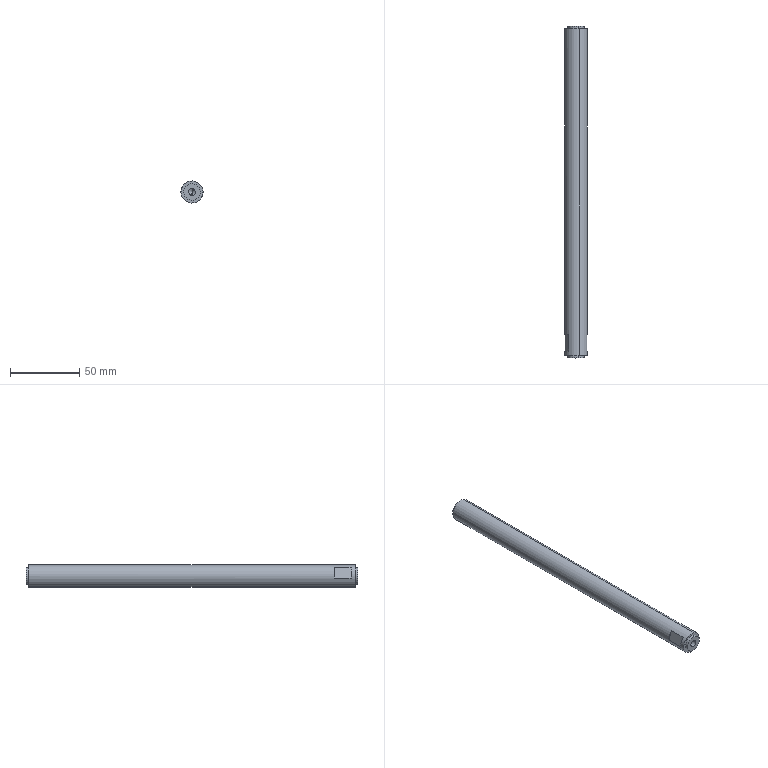Component | SolidWorks | F01AE00111-A2014-1 | 1 solid | 24 faces | box 16 x 240 x 16 mm | volume 47169 mm3 | cylinder 10 | plane 10 | cone 4 | commonest cylinder face diameters 5 x4 12 x4 16 x2 | material Hard Chrome Plated Rod
build123d program:
from build123d import *

# Parameters (mm, degrees)
SKETCH1_R             = 8
BOSS_EXTRUDE1_DEPTH   = 240
CHAMFER1_SIZE         = 1
M6_TAPPED_HOLE1_D     = 5
M6_TAPPED_HOLE1_DEPTH = 15
M6_TAPPED_HOLE1_TIP   = 1.502
SKETCH4_R             = 10.068
SKETCH4_R_2           = 6
CUT_EXTRUDE1_DEPTH    = 2
M6_TAPPED_HOLE2_D     = 5
M6_TAPPED_HOLE2_DEPTH = 15
M6_TAPPED_HOLE2_TIP   = 1.502
SKETCH7_W             = 3.867
SKETCH7_H             = 17.751
SKETCH7_W_2           = 7.143
SKETCH7_H_2           = 17.096
CUT_EXTRUDE2_DEPTH    = 12
SKETCH8_OUTSIDE_W     = 66.212
SKETCH8_OUTSIDE_H     = 66.212
SKETCH8_OUTSIDE_R     = 6
CUT_EXTRUDE3_DEPTH    = 2


with BuildPart() as part:
    # Sketch1 → Boss-Extrude1 (new body)
    with BuildSketch(Plane(origin=(0, 0, 0), x_dir=(1, 0, 0), z_dir=(0, 1, 0))):
        with Locations(Location((0, 0, 0), (0, 0, 270))):
            Circle(SKETCH1_R)
    extrude(amount=BOSS_EXTRUDE1_DEPTH)

    # Chamfer1
    chamfer1_edges = [part.edges().sort_by_distance(p)[0] for p in [
        (0, 0, -8),
        (0, 240, -8),
    ]]
    chamfer(chamfer1_edges, length=CHAMFER1_SIZE)

    # M6 Tapped Hole1
    with Locations(Plane(origin=(0, 240, 0), x_dir=(1, 0, 0), z_dir=(0, 1, 0))):
        with Locations((0, 0)):
            Hole(M6_TAPPED_HOLE1_D / 2, depth=M6_TAPPED_HOLE1_DEPTH)
            with Locations((0, 0, -(M6_TAPPED_HOLE1_DEPTH + M6_TAPPED_HOLE1_TIP / 2))):  # 118° drill point
                Cone(0, M6_TAPPED_HOLE1_D / 2, M6_TAPPED_HOLE1_TIP, mode=Mode.SUBTRACT)

    # Sketch4 → Cut-Extrude1 (cut)
    with BuildSketch(Plane(origin=(0, 240, 0), x_dir=(1, 0, 0), z_dir=(0, 1, 0))):
        Circle(SKETCH4_R)
        with Locations(Location((0, 0, 0), (0, 0, 270))):
            Circle(SKETCH4_R_2, mode=Mode.SUBTRACT)
    extrude(amount=-CUT_EXTRUDE1_DEPTH, mode=Mode.SUBTRACT)

    # M6 Tapped Hole2
    with Locations(Plane(origin=(0, 0, 0), x_dir=(-1, 0, 0), z_dir=(0, -1, 0))):
        with Locations((0, 0)):
            Hole(M6_TAPPED_HOLE2_D / 2, depth=M6_TAPPED_HOLE2_DEPTH)
            with Locations((0, 0, -(M6_TAPPED_HOLE2_DEPTH + M6_TAPPED_HOLE2_TIP / 2))):  # 118° drill point
                Cone(0, M6_TAPPED_HOLE2_D / 2, M6_TAPPED_HOLE2_TIP, mode=Mode.SUBTRACT)

    # Sketch7 → Cut-Extrude2 (cut)
    with BuildSketch(Plane(origin=(0, 5, 0), x_dir=(-1, 0, 0), z_dir=(0, -1, 0))):
        with Locations((-8.934, -0.05283)):
            Rectangle(SKETCH7_W, SKETCH7_H)
        with Locations((10.571, -0.2958)):
            Rectangle(SKETCH7_W_2, SKETCH7_H_2)
    extrude(amount=-CUT_EXTRUDE2_DEPTH, mode=Mode.SUBTRACT)

    # Sketch8 outside → Cut-Extrude3 (cut)
    with BuildSketch(Plane.XZ):
        Rectangle(SKETCH8_OUTSIDE_W, SKETCH8_OUTSIDE_H)
        with Locations(Location((0, 0, 0), (0, 0, 90))):
            Circle(SKETCH8_OUTSIDE_R, mode=Mode.SUBTRACT)
    extrude(amount=-CUT_EXTRUDE3_DEPTH, mode=Mode.SUBTRACT)


solid = part.part

# Placed as in the assembly
solid = solid.moved(Location((-84.852, -192.452, -211.475), (0, 18.481, 0)))
STEP:
#1=CARTESIAN_POINT('',(-3.309,-6.986,-8.232));
#2=VERTEX_POINT('',#1);
#3=CARTESIAN_POINT('',(-3.372,-6.986,-8.419));
#4=VERTEX_POINT('',#3);
#5=CARTESIAN_POINT('',(-3.341,-6.986,-8.326));
#6=DIRECTION('',(0.,-1.,0.));
#7=DIRECTION('',(-0.317,0.,-0.9484));
#8=AXIS2_PLACEMENT_3D('',#5,#6,#7);
#9=CIRCLE('',#8,0.09843);
#10=EDGE_CURVE('',#2,#4,#9,.T.);
#11=ORIENTED_EDGE('',*,*,#10,.F.);
#12=CARTESIAN_POINT('',(-3.309,-7.577,-8.232));
#13=VERTEX_POINT('',#12);
#14=CARTESIAN_POINT('',(-3.309,-7.577,-8.232));
#15=DIRECTION('',(0.,-1.,0.));
#16=VECTOR('',#15,39.37);
#17=LINE('',#14,#16);
#18=EDGE_CURVE('',#2,#13,#17,.T.);
#19=ORIENTED_EDGE('',*,*,#18,.T.);
#20=CARTESIAN_POINT('',(-3.372,-7.577,-8.419));
#21=VERTEX_POINT('',#20);
#22=CARTESIAN_POINT('',(-3.341,-7.577,-8.326));
#23=DIRECTION('',(0.,-1.,0.));
#24=DIRECTION('',(-0.317,0.,-0.9484));
#25=AXIS2_PLACEMENT_3D('',#22,#23,#24);
#26=CIRCLE('',#25,0.09843);
#27=EDGE_CURVE('',#13,#21,#26,.T.);
#28=ORIENTED_EDGE('',*,*,#27,.T.);
#29=CARTESIAN_POINT('',(-3.372,-7.577,-8.419));
#30=DIRECTION('',(0.,-1.,0.));
#31=VECTOR('',#30,39.37);
#32=LINE('',#29,#31);
#33=EDGE_CURVE('',#4,#21,#32,.T.);
#34=ORIENTED_EDGE('',*,*,#33,.F.);
#35=EDGE_LOOP('',(#11,#19,#28,#34));
#36=FACE_OUTER_BOUND('',#35,.T.);
#37=CARTESIAN_POINT('',(-3.341,-7.577,-8.326));
#38=DIRECTION('',(0.,-1.,0.));
#39=DIRECTION('',(-0.317,0.,-0.9484));
#40=AXIS2_PLACEMENT_3D('',#37,#38,#39);
#41=CYLINDRICAL_SURFACE('',#40,0.09843);
#42=ADVANCED_FACE('',(#36),#41,.F.);
#43=CARTESIAN_POINT('',(-3.341,-6.927,-8.326));
#44=VERTEX_POINT('',#43);
#45=CARTESIAN_POINT('',(-3.372,-6.986,-8.419));
#46=DIRECTION('',(-0.2717,-0.515,-0.813));
#47=VECTOR('',#46,39.37);
#48=LINE('',#45,#47);
#49=EDGE_CURVE('',#44,#4,#48,.T.);
#50=ORIENTED_EDGE('',*,*,#49,.F.);
#51=CARTESIAN_POINT('',(-3.309,-6.986,-8.232));
#52=DIRECTION('',(0.2717,-0.515,0.813));
#53=VECTOR('',#52,39.37);
#54=LINE('',#51,#53);
#55=EDGE_CURVE('',#44,#2,#54,.T.);
#56=ORIENTED_EDGE('',*,*,#55,.T.);
#57=ORIENTED_EDGE('',*,*,#10,.T.);
#58=EDGE_LOOP('',(#50,#56,#57));
#59=FACE_OUTER_BOUND('',#58,.T.);
#60=CARTESIAN_POINT('',(-3.341,-6.986,-8.326));
#61=DIRECTION('',(0.,-1.,0.));
#62=DIRECTION('',(-0.317,0.,-0.9484));
#63=AXIS2_PLACEMENT_3D('',#60,#61,#62);
#64=CONICAL_SURFACE('',#63,0.09843,1.03);
#65=ADVANCED_FACE('',(#59),#64,.F.);
#66=CARTESIAN_POINT('',(-3.416,-7.498,-8.55));
#67=VERTEX_POINT('',#66);
#68=CARTESIAN_POINT('',(-3.266,-7.498,-8.102));
#69=VERTEX_POINT('',#68);
#70=CARTESIAN_POINT('',(-3.341,-7.498,-8.326));
#71=DIRECTION('',(0.,-1.,0.));
#72=DIRECTION('',(-0.317,0.,-0.9484));
#73=AXIS2_PLACEMENT_3D('',#70,#71,#72);
#74=CIRCLE('',#73,0.2362);
#75=EDGE_CURVE('',#67,#69,#74,.T.);
#76=ORIENTED_EDGE('',*,*,#75,.T.);
#77=CARTESIAN_POINT('',(-3.266,-7.577,-8.102));
#78=VERTEX_POINT('',#77);
#79=CARTESIAN_POINT('',(-3.266,-7.498,-8.102));
#80=DIRECTION('',(0.,-1.,0.));
#81=VECTOR('',#80,39.37);
#82=LINE('',#79,#81);
#83=EDGE_CURVE('',#69,#78,#82,.T.);
#84=ORIENTED_EDGE('',*,*,#83,.T.);
#85=CARTESIAN_POINT('',(-3.416,-7.577,-8.55));
#86=VERTEX_POINT('',#85);
#87=CARTESIAN_POINT('',(-3.341,-7.577,-8.326));
#88=DIRECTION('',(0.,-1.,0.));
#89=DIRECTION('',(-0.317,0.,-0.9484));
#90=AXIS2_PLACEMENT_3D('',#87,#88,#89);
#91=CIRCLE('',#90,0.2362);
#92=EDGE_CURVE('',#86,#78,#91,.T.);
#93=ORIENTED_EDGE('',*,*,#92,.F.);
#94=CARTESIAN_POINT('',(-3.416,-7.498,-8.55));
#95=DIRECTION('',(0.,-1.,0.));
#96=VECTOR('',#95,39.37);
#97=LINE('',#94,#96);
#98=EDGE_CURVE('',#67,#86,#97,.T.);
#99=ORIENTED_EDGE('',*,*,#98,.F.);
#100=EDGE_LOOP('',(#76,#84,#93,#99));
#101=FACE_OUTER_BOUND('',#100,.T.);
#102=CARTESIAN_POINT('',(-3.341,-7.498,-8.326));
#103=DIRECTION('',(0.,-1.,0.));
#104=DIRECTION('',(-0.317,0.,-0.9484));
#105=AXIS2_PLACEMENT_3D('',#102,#103,#104);
#106=CYLINDRICAL_SURFACE('',#105,0.2362);
#107=ADVANCED_FACE('',(#101),#106,.T.);
#108=CARTESIAN_POINT('',(-3.372,1.281,-8.419));
#109=VERTEX_POINT('',#108);
#110=CARTESIAN_POINT('',(-3.309,1.281,-8.232));
#111=VERTEX_POINT('',#110);
#112=CARTESIAN_POINT('',(-3.341,1.281,-8.326));
#113=DIRECTION('',(0.,1.,0.));
#114=DIRECTION('',(0.317,0.,0.9484));
#115=AXIS2_PLACEMENT_3D('',#112,#113,#114);
#116=CIRCLE('',#115,0.09843);
#117=EDGE_CURVE('',#109,#111,#116,.T.);
#118=ORIENTED_EDGE('',*,*,#117,.F.);
#119=CARTESIAN_POINT('',(-3.372,1.872,-8.419));
#120=VERTEX_POINT('',#119);
#121=CARTESIAN_POINT('',(-3.372,1.872,-8.419));
#122=DIRECTION('',(0.,1.,0.));
#123=VECTOR('',#122,39.37);
#124=LINE('',#121,#123);
#125=EDGE_CURVE('',#109,#120,#124,.T.);
#126=ORIENTED_EDGE('',*,*,#125,.T.);
#127=CARTESIAN_POINT('',(-3.309,1.872,-8.232));
#128=VERTEX_POINT('',#127);
#129=CARTESIAN_POINT('',(-3.341,1.872,-8.326));
#130=DIRECTION('',(0.,1.,0.));
#131=DIRECTION('',(0.317,0.,0.9484));
#132=AXIS2_PLACEMENT_3D('',#129,#130,#131);
#133=CIRCLE('',#132,0.09843);
#134=EDGE_CURVE('',#120,#128,#133,.T.);
#135=ORIENTED_EDGE('',*,*,#134,.T.);
#136=CARTESIAN_POINT('',(-3.309,1.872,-8.232));
#137=DIRECTION('',(0.,1.,0.));
#138=VECTOR('',#137,39.37);
#139=LINE('',#136,#138);
#140=EDGE_CURVE('',#111,#128,#139,.T.);
#141=ORIENTED_EDGE('',*,*,#140,.F.);
#142=EDGE_LOOP('',(#118,#126,#135,#141));
#143=FACE_OUTER_BOUND('',#142,.T.);
#144=CARTESIAN_POINT('',(-3.341,1.872,-8.326));
#145=DIRECTION('',(0.,1.,0.));
#146=DIRECTION('',(0.317,0.,0.9484));
#147=AXIS2_PLACEMENT_3D('',#144,#145,#146);
#148=CYLINDRICAL_SURFACE('',#147,0.09843);
#149=ADVANCED_FACE('',(#143),#148,.F.);
#150=CARTESIAN_POINT('',(-3.341,1.222,-8.326));
#151=VERTEX_POINT('',#150);
#152=CARTESIAN_POINT('',(-3.309,1.281,-8.232));
#153=DIRECTION('',(0.2717,0.515,0.813));
#154=VECTOR('',#153,39.37);
#155=LINE('',#152,#154);
#156=EDGE_CURVE('',#151,#111,#155,.T.);
#157=ORIENTED_EDGE('',*,*,#156,.F.);
#158=CARTESIAN_POINT('',(-3.372,1.281,-8.419));
#159=DIRECTION('',(-0.2717,0.515,-0.813));
#160=VECTOR('',#159,39.37);
#161=LINE('',#158,#160);
#162=EDGE_CURVE('',#151,#109,#161,.T.);
#163=ORIENTED_EDGE('',*,*,#162,.T.);
#164=ORIENTED_EDGE('',*,*,#117,.T.);
#165=EDGE_LOOP('',(#157,#163,#164));
#166=FACE_OUTER_BOUND('',#165,.T.);
#167=CARTESIAN_POINT('',(-3.341,1.281,-8.326));
#168=DIRECTION('',(0.,1.,0.));
#169=DIRECTION('',(0.317,0.,0.9484));
#170=AXIS2_PLACEMENT_3D('',#167,#168,#169);
#171=CONICAL_SURFACE('',#170,0.09843,1.03);
#172=ADVANCED_FACE('',(#166),#171,.F.);
#173=CARTESIAN_POINT('',(-3.266,1.793,-8.102));
#174=VERTEX_POINT('',#173);
#175=CARTESIAN_POINT('',(-3.416,1.793,-8.55));
#176=VERTEX_POINT('',#175);
#177=CARTESIAN_POINT('',(-3.341,1.793,-8.326));
#178=DIRECTION('',(0.,1.,0.));
#179=DIRECTION('',(0.317,0.,0.9484));
#180=AXIS2_PLACEMENT_3D('',#177,#178,#179);
#181=CIRCLE('',#180,0.2362);
#182=EDGE_CURVE('',#174,#176,#181,.T.);
#183=ORIENTED_EDGE('',*,*,#182,.T.);
#184=CARTESIAN_POINT('',(-3.416,1.872,-8.55));
#185=VERTEX_POINT('',#184);
#186=CARTESIAN_POINT('',(-3.416,1.793,-8.55));
#187=DIRECTION('',(0.,1.,0.));
#188=VECTOR('',#187,39.37);
#189=LINE('',#186,#188);
#190=EDGE_CURVE('',#176,#185,#189,.T.);
#191=ORIENTED_EDGE('',*,*,#190,.T.);
#192=CARTESIAN_POINT('',(-3.266,1.872,-8.102));
#193=VERTEX_POINT('',#192);
#194=CARTESIAN_POINT('',(-3.341,1.872,-8.326));
#195=DIRECTION('',(0.,1.,0.));
#196=DIRECTION('',(0.317,0.,0.9484));
#197=AXIS2_PLACEMENT_3D('',#194,#195,#196);
#198=CIRCLE('',#197,0.2362);
#199=EDGE_CURVE('',#193,#185,#198,.T.);
#200=ORIENTED_EDGE('',*,*,#199,.F.);
#201=CARTESIAN_POINT('',(-3.266,1.793,-8.102));
#202=DIRECTION('',(0.,1.,0.));
#203=VECTOR('',#202,39.37);
#204=LINE('',#201,#203);
#205=EDGE_CURVE('',#174,#193,#204,.T.);
#206=ORIENTED_EDGE('',*,*,#205,.F.);
#207=EDGE_LOOP('',(#183,#191,#200,#206));
#208=FACE_OUTER_BOUND('',#207,.T.);
#209=CARTESIAN_POINT('',(-3.341,1.793,-8.326));
#210=DIRECTION('',(0.,1.,0.));
#211=DIRECTION('',(0.317,0.,0.9484));
#212=AXIS2_PLACEMENT_3D('',#209,#210,#211);
#213=CYLINDRICAL_SURFACE('',#212,0.2362);
#214=ADVANCED_FACE('',(#208),#213,.T.);
#215=CARTESIAN_POINT('',(-3.128,-6.908,-8.558));
#216=VERTEX_POINT('',#215);
#217=CARTESIAN_POINT('',(-3.031,-6.908,-8.269));
#218=VERTEX_POINT('',#217);
#219=CARTESIAN_POINT('',(-3.341,-6.908,-8.326));
#220=DIRECTION('',(0.,-1.,0.));
#221=DIRECTION('',(-0.317,0.,-0.9484));
#222=AXIS2_PLACEMENT_3D('',#219,#220,#221);
#223=CIRCLE('',#222,0.315);
#224=EDGE_CURVE('',#216,#218,#223,.T.);
#225=ORIENTED_EDGE('',*,*,#224,.F.);
#226=CARTESIAN_POINT('',(-3.128,-7.38,-8.558));
#227=VERTEX_POINT('',#226);
#228=CARTESIAN_POINT('',(-3.128,1.872,-8.558));
#229=DIRECTION('',(0.,-1.,0.));
#230=VECTOR('',#229,39.37);
#231=LINE('',#228,#230);
#232=EDGE_CURVE('',#216,#227,#231,.T.);
#233=ORIENTED_EDGE('',*,*,#232,.T.);
#234=CARTESIAN_POINT('',(-3.031,-7.38,-8.269));
#235=VERTEX_POINT('',#234);
#236=CARTESIAN_POINT('',(-3.341,-7.38,-8.326));
#237=DIRECTION('',(0.,-1.,0.));
#238=DIRECTION('',(-0.317,0.,-0.9484));
#239=AXIS2_PLACEMENT_3D('',#236,#237,#238);
#240=CIRCLE('',#239,0.315);
#241=EDGE_CURVE('',#227,#235,#240,.T.);
#242=ORIENTED_EDGE('',*,*,#241,.T.);
#243=CARTESIAN_POINT('',(-3.031,1.872,-8.269));
#244=DIRECTION('',(0.,1.,0.));
#245=VECTOR('',#244,39.37);
#246=LINE('',#243,#245);
#247=EDGE_CURVE('',#235,#218,#246,.T.);
#248=ORIENTED_EDGE('',*,*,#247,.T.);
#249=EDGE_LOOP('',(#225,#233,#242,#248));
#250=FACE_BOUND('',#249,.T.);
#251=CARTESIAN_POINT('',(-3.241,1.793,-8.027));
#252=VERTEX_POINT('',#251);
#253=CARTESIAN_POINT('',(-3.44,1.793,-8.624));
#254=VERTEX_POINT('',#253);
#255=CARTESIAN_POINT('',(-3.341,1.793,-8.326));
#256=DIRECTION('',(0.,1.,0.));
#257=DIRECTION('',(0.317,0.,0.9484));
#258=AXIS2_PLACEMENT_3D('',#255,#256,#257);
#259=CIRCLE('',#258,0.315);
#260=EDGE_CURVE('',#252,#254,#259,.T.);
#261=ORIENTED_EDGE('',*,*,#260,.F.);
#262=CARTESIAN_POINT('',(-3.241,-7.498,-8.027));
#263=VERTEX_POINT('',#262);
#264=CARTESIAN_POINT('',(-3.241,1.872,-8.027));
#265=DIRECTION('',(0.,-1.,0.));
#266=VECTOR('',#265,39.37);
#267=LINE('',#264,#266);
#268=EDGE_CURVE('',#252,#263,#267,.T.);
#269=ORIENTED_EDGE('',*,*,#268,.T.);
#270=CARTESIAN_POINT('',(-3.44,-7.498,-8.624));
#271=VERTEX_POINT('',#270);
#272=CARTESIAN_POINT('',(-3.341,-7.498,-8.326));
#273=DIRECTION('',(0.,-1.,0.));
#274=DIRECTION('',(-0.317,0.,-0.9484));
#275=AXIS2_PLACEMENT_3D('',#272,#273,#274);
#276=CIRCLE('',#275,0.315);
#277=EDGE_CURVE('',#271,#263,#276,.T.);
#278=ORIENTED_EDGE('',*,*,#277,.F.);
#279=CARTESIAN_POINT('',(-3.44,1.872,-8.624));
#280=DIRECTION('',(0.,-1.,0.));
#281=VECTOR('',#280,39.37);
#282=LINE('',#279,#281);
#283=EDGE_CURVE('',#254,#271,#282,.T.);
#284=ORIENTED_EDGE('',*,*,#283,.F.);
#285=EDGE_LOOP('',(#261,#269,#278,#284));
#286=FACE_OUTER_BOUND('',#285,.T.);
#287=CARTESIAN_POINT('',(-3.341,1.872,-8.326));
#288=DIRECTION('',(0.,-1.,0.));
#289=DIRECTION('',(-0.317,0.,-0.9484));
#290=AXIS2_PLACEMENT_3D('',#287,#288,#289);
#291=CYLINDRICAL_SURFACE('',#290,0.315);
#292=ADVANCED_FACE('',(#250,#286),#291,.T.);
#293=ORIENTED_EDGE('',*,*,#268,.F.);
#294=CARTESIAN_POINT('',(-3.341,1.793,-8.326));
#295=DIRECTION('',(0.,1.,0.));
#296=DIRECTION('',(0.317,0.,0.9484));
#297=AXIS2_PLACEMENT_3D('',#294,#295,#296);
#298=CIRCLE('',#297,0.315);
#299=EDGE_CURVE('',#254,#252,#298,.T.);
#300=ORIENTED_EDGE('',*,*,#299,.F.);
#301=ORIENTED_EDGE('',*,*,#283,.T.);
#302=CARTESIAN_POINT('',(-3.341,-7.498,-8.326));
#303=DIRECTION('',(0.,-1.,0.));
#304=DIRECTION('',(-0.317,0.,-0.9484));
#305=AXIS2_PLACEMENT_3D('',#302,#303,#304);
#306=CIRCLE('',#305,0.315);
#307=EDGE_CURVE('',#263,#271,#306,.T.);
#308=ORIENTED_EDGE('',*,*,#307,.F.);
#309=EDGE_LOOP('',(#293,#300,#301,#308));
#310=FACE_OUTER_BOUND('',#309,.T.);
#311=CARTESIAN_POINT('',(-3.554,-6.908,-8.094));
#312=VERTEX_POINT('',#311);
#313=CARTESIAN_POINT('',(-3.65,-6.908,-8.383));
#314=VERTEX_POINT('',#313);
#315=CARTESIAN_POINT('',(-3.341,-6.908,-8.326));
#316=DIRECTION('',(0.,-1.,0.));
#317=DIRECTION('',(-0.317,0.,-0.9484));
#318=AXIS2_PLACEMENT_3D('',#315,#316,#317);
#319=CIRCLE('',#318,0.315);
#320=EDGE_CURVE('',#312,#314,#319,.T.);
#321=ORIENTED_EDGE('',*,*,#320,.F.);
#322=CARTESIAN_POINT('',(-3.554,-7.38,-8.094));
#323=VERTEX_POINT('',#322);
#324=CARTESIAN_POINT('',(-3.554,1.872,-8.094));
#325=DIRECTION('',(0.,-1.,0.));
#326=VECTOR('',#325,39.37);
#327=LINE('',#324,#326);
#328=EDGE_CURVE('',#312,#323,#327,.T.);
#329=ORIENTED_EDGE('',*,*,#328,.T.);
#330=CARTESIAN_POINT('',(-3.65,-7.38,-8.383));
#331=VERTEX_POINT('',#330);
#332=CARTESIAN_POINT('',(-3.341,-7.38,-8.326));
#333=DIRECTION('',(0.,-1.,0.));
#334=DIRECTION('',(-0.317,0.,-0.9484));
#335=AXIS2_PLACEMENT_3D('',#332,#333,#334);
#336=CIRCLE('',#335,0.315);
#337=EDGE_CURVE('',#323,#331,#336,.T.);
#338=ORIENTED_EDGE('',*,*,#337,.T.);
#339=CARTESIAN_POINT('',(-3.65,1.872,-8.383));
#340=DIRECTION('',(0.,1.,0.));
#341=VECTOR('',#340,39.37);
#342=LINE('',#339,#341);
#343=EDGE_CURVE('',#331,#314,#342,.T.);
#344=ORIENTED_EDGE('',*,*,#343,.T.);
#345=EDGE_LOOP('',(#321,#329,#338,#344));
#346=FACE_BOUND('',#345,.T.);
#347=CARTESIAN_POINT('',(-3.341,1.872,-8.326));
#348=DIRECTION('',(0.,-1.,0.));
#349=DIRECTION('',(-0.317,0.,-0.9484));
#350=AXIS2_PLACEMENT_3D('',#347,#348,#349);
#351=CYLINDRICAL_SURFACE('',#350,0.315);
#352=ADVANCED_FACE('',(#310,#346),#351,.T.);
#353=ORIENTED_EDGE('',*,*,#182,.F.);
#354=CARTESIAN_POINT('',(-3.341,1.793,-8.326));
#355=DIRECTION('',(0.,1.,0.));
#356=DIRECTION('',(0.317,0.,0.9484));
#357=AXIS2_PLACEMENT_3D('',#354,#355,#356);
#358=CIRCLE('',#357,0.2362);
#359=EDGE_CURVE('',#176,#174,#358,.T.);
#360=ORIENTED_EDGE('',*,*,#359,.F.);
#361=EDGE_LOOP('',(#353,#360));
#362=FACE_BOUND('',#361,.T.);
#363=ORIENTED_EDGE('',*,*,#299,.T.);
#364=ORIENTED_EDGE('',*,*,#260,.T.);
#365=EDGE_LOOP('',(#363,#364));
#366=FACE_OUTER_BOUND('',#365,.T.);
#367=CARTESIAN_POINT('',(-3.341,1.793,-8.326));
#368=DIRECTION('',(0.,1.,0.));
#369=DIRECTION('',(0.317,0.,0.9484));
#370=AXIS2_PLACEMENT_3D('',#367,#368,#369);
#371=PLANE('',#370);
#372=ADVANCED_FACE('',(#362,#366),#371,.T.);
#373=ORIENTED_EDGE('',*,*,#190,.F.);
#374=ORIENTED_EDGE('',*,*,#359,.T.);
#375=ORIENTED_EDGE('',*,*,#205,.T.);
#376=CARTESIAN_POINT('',(-3.341,1.872,-8.326));
#377=DIRECTION('',(0.,1.,0.));
#378=DIRECTION('',(0.317,0.,0.9484));
#379=AXIS2_PLACEMENT_3D('',#376,#377,#378);
#380=CIRCLE('',#379,0.2362);
#381=EDGE_CURVE('',#185,#193,#380,.T.);
#382=ORIENTED_EDGE('',*,*,#381,.F.);
#383=EDGE_LOOP('',(#373,#374,#375,#382));
#384=FACE_OUTER_BOUND('',#383,.T.);
#385=CARTESIAN_POINT('',(-3.341,1.793,-8.326));
#386=DIRECTION('',(0.,1.,0.));
#387=DIRECTION('',(0.317,0.,0.9484));
#388=AXIS2_PLACEMENT_3D('',#385,#386,#387);
#389=CYLINDRICAL_SURFACE('',#388,0.2362);
#390=ADVANCED_FACE('',(#384),#389,.T.);
#391=ORIENTED_EDGE('',*,*,#162,.F.);
#392=ORIENTED_EDGE('',*,*,#156,.T.);
#393=CARTESIAN_POINT('',(-3.341,1.281,-8.326));
#394=DIRECTION('',(0.,1.,0.));
#395=DIRECTION('',(0.317,0.,0.9484));
#396=AXIS2_PLACEMENT_3D('',#393,#394,#395);
#397=CIRCLE('',#396,0.09843);
#398=EDGE_CURVE('',#111,#109,#397,.T.);
#399=ORIENTED_EDGE('',*,*,#398,.T.);
#400=EDGE_LOOP('',(#391,#392,#399));
#401=FACE_OUTER_BOUND('',#400,.T.);
#402=CARTESIAN_POINT('',(-3.341,1.281,-8.326));
#403=DIRECTION('',(0.,1.,0.));
#404=DIRECTION('',(0.317,0.,0.9484));
#405=AXIS2_PLACEMENT_3D('',#402,#403,#404);
#406=CONICAL_SURFACE('',#405,0.09843,1.03);
#407=ADVANCED_FACE('',(#401),#406,.F.);
#408=ORIENTED_EDGE('',*,*,#125,.F.);
#409=ORIENTED_EDGE('',*,*,#398,.F.);
#410=ORIENTED_EDGE('',*,*,#140,.T.);
#411=CARTESIAN_POINT('',(-3.341,1.872,-8.326));
#412=DIRECTION('',(0.,1.,0.));
#413=DIRECTION('',(0.317,0.,0.9484));
#414=AXIS2_PLACEMENT_3D('',#411,#412,#413);
#415=CIRCLE('',#414,0.09843);
#416=EDGE_CURVE('',#128,#120,#415,.T.);
#417=ORIENTED_EDGE('',*,*,#416,.T.);
#418=EDGE_LOOP('',(#408,#409,#410,#417));
#419=FACE_OUTER_BOUND('',#418,.T.);
#420=CARTESIAN_POINT('',(-3.341,1.872,-8.326));
#421=DIRECTION('',(0.,1.,0.));
#422=DIRECTION('',(0.317,0.,0.9484));
#423=AXIS2_PLACEMENT_3D('',#420,#421,#422);
#424=CYLINDRICAL_SURFACE('',#423,0.09843);
#425=ADVANCED_FACE('',(#419),#424,.F.);
#426=ORIENTED_EDGE('',*,*,#416,.F.);
#427=ORIENTED_EDGE('',*,*,#134,.F.);
#428=EDGE_LOOP('',(#426,#427));
#429=FACE_BOUND('',#428,.T.);
#430=ORIENTED_EDGE('',*,*,#199,.T.);
#431=ORIENTED_EDGE('',*,*,#381,.T.);
#432=EDGE_LOOP('',(#430,#431));
#433=FACE_OUTER_BOUND('',#432,.T.);
#434=CARTESIAN_POINT('',(-3.341,1.872,-8.326));
#435=DIRECTION('',(0.,1.,0.));
#436=DIRECTION('',(0.317,0.,0.9484));
#437=AXIS2_PLACEMENT_3D('',#434,#435,#436);
#438=PLANE('',#437);
#439=ADVANCED_FACE('',(#429,#433),#438,.T.);
#440=CARTESIAN_POINT('',(-3.189,-6.908,-8.743));
#441=DIRECTION('',(-0.317,0.,-0.9484));
#442=VECTOR('',#441,39.37);
#443=LINE('',#440,#442);
#444=EDGE_CURVE('',#218,#216,#443,.T.);
#445=ORIENTED_EDGE('',*,*,#444,.F.);
#446=ORIENTED_EDGE('',*,*,#247,.F.);
#447=CARTESIAN_POINT('',(-3.189,-7.38,-8.743));
#448=DIRECTION('',(-0.317,0.,-0.9484));
#449=VECTOR('',#448,39.37);
#450=LINE('',#447,#449);
#451=EDGE_CURVE('',#235,#227,#450,.T.);
#452=ORIENTED_EDGE('',*,*,#451,.T.);
#453=ORIENTED_EDGE('',*,*,#232,.F.);
#454=EDGE_LOOP('',(#445,#446,#452,#453));
#455=FACE_OUTER_BOUND('',#454,.T.);
#456=CARTESIAN_POINT('',(-3.189,-6.908,-8.743));
#457=DIRECTION('',(-0.9484,0.,0.317));
#458=DIRECTION('',(0.317,0.,0.9484));
#459=AXIS2_PLACEMENT_3D('',#456,#457,#458);
#460=PLANE('',#459);
#461=ADVANCED_FACE('',(#455),#460,.F.);
#462=ORIENTED_EDGE('',*,*,#224,.T.);
#463=ORIENTED_EDGE('',*,*,#444,.T.);
#464=EDGE_LOOP('',(#462,#463));
#465=FACE_OUTER_BOUND('',#464,.T.);
#466=CARTESIAN_POINT('',(-3.341,-6.908,-8.326));
#467=DIRECTION('',(0.,-1.,0.));
#468=DIRECTION('',(-0.317,0.,-0.9484));
#469=AXIS2_PLACEMENT_3D('',#466,#467,#468);
#470=PLANE('',#469);
#471=ADVANCED_FACE('',(#465),#470,.T.);
#472=ORIENTED_EDGE('',*,*,#451,.F.);
#473=ORIENTED_EDGE('',*,*,#241,.F.);
#474=EDGE_LOOP('',(#472,#473));
#475=FACE_OUTER_BOUND('',#474,.T.);
#476=CARTESIAN_POINT('',(-3.341,-7.38,-8.326));
#477=DIRECTION('',(0.,-1.,0.));
#478=DIRECTION('',(-0.317,0.,-0.9484));
#479=AXIS2_PLACEMENT_3D('',#476,#477,#478);
#480=PLANE('',#479);
#481=ADVANCED_FACE('',(#475),#480,.F.);
#482=CARTESIAN_POINT('',(-3.705,-6.908,-8.547));
#483=DIRECTION('',(0.317,0.,0.9484));
#484=VECTOR('',#483,39.37);
#485=LINE('',#482,#484);
#486=EDGE_CURVE('',#314,#312,#485,.T.);
#487=ORIENTED_EDGE('',*,*,#486,.F.);
#488=ORIENTED_EDGE('',*,*,#343,.F.);
#489=CARTESIAN_POINT('',(-3.705,-7.38,-8.547));
#490=DIRECTION('',(0.317,0.,0.9484));
#491=VECTOR('',#490,39.37);
#492=LINE('',#489,#491);
#493=EDGE_CURVE('',#331,#323,#492,.T.);
#494=ORIENTED_EDGE('',*,*,#493,.T.);
#495=ORIENTED_EDGE('',*,*,#328,.F.);
#496=EDGE_LOOP('',(#487,#488,#494,#495));
#497=FACE_OUTER_BOUND('',#496,.T.);
#498=CARTESIAN_POINT('',(-3.705,-6.908,-8.547));
#499=DIRECTION('',(0.9484,0.,-0.317));
#500=DIRECTION('',(-0.317,0.,-0.9484));
#501=AXIS2_PLACEMENT_3D('',#498,#499,#500);
#502=PLANE('',#501);
#503=ADVANCED_FACE('',(#497),#502,.F.);
#504=ORIENTED_EDGE('',*,*,#320,.T.);
#505=ORIENTED_EDGE('',*,*,#486,.T.);
#506=EDGE_LOOP('',(#504,#505));
#507=FACE_OUTER_BOUND('',#506,.T.);
#508=CARTESIAN_POINT('',(-3.341,-6.908,-8.326));
#509=DIRECTION('',(0.,-1.,0.));
#510=DIRECTION('',(-0.317,0.,-0.9484));
#511=AXIS2_PLACEMENT_3D('',#508,#509,#510);
#512=PLANE('',#511);
#513=ADVANCED_FACE('',(#507),#512,.T.);
#514=ORIENTED_EDGE('',*,*,#493,.F.);
#515=ORIENTED_EDGE('',*,*,#337,.F.);
#516=EDGE_LOOP('',(#514,#515));
#517=FACE_OUTER_BOUND('',#516,.T.);
#518=CARTESIAN_POINT('',(-3.341,-7.38,-8.326));
#519=DIRECTION('',(0.,-1.,0.));
#520=DIRECTION('',(-0.317,0.,-0.9484));
#521=AXIS2_PLACEMENT_3D('',#518,#519,#520);
#522=PLANE('',#521);
#523=ADVANCED_FACE('',(#517),#522,.F.);
#524=ORIENTED_EDGE('',*,*,#75,.F.);
#525=CARTESIAN_POINT('',(-3.341,-7.498,-8.326));
#526=DIRECTION('',(0.,-1.,0.));
#527=DIRECTION('',(-0.317,0.,-0.9484));
#528=AXIS2_PLACEMENT_3D('',#525,#526,#527);
#529=CIRCLE('',#528,0.2362);
#530=EDGE_CURVE('',#69,#67,#529,.T.);
#531=ORIENTED_EDGE('',*,*,#530,.F.);
#532=EDGE_LOOP('',(#524,#531));
#533=FACE_BOUND('',#532,.T.);
#534=ORIENTED_EDGE('',*,*,#277,.T.);
#535=ORIENTED_EDGE('',*,*,#307,.T.);
#536=EDGE_LOOP('',(#534,#535));
#537=FACE_OUTER_BOUND('',#536,.T.);
#538=CARTESIAN_POINT('',(-3.341,-7.498,-8.326));
#539=DIRECTION('',(0.,-1.,0.));
#540=DIRECTION('',(-0.317,0.,-0.9484));
#541=AXIS2_PLACEMENT_3D('',#538,#539,#540);
#542=PLANE('',#541);
#543=ADVANCED_FACE('',(#533,#537),#542,.T.);
#544=ORIENTED_EDGE('',*,*,#83,.F.);
#545=ORIENTED_EDGE('',*,*,#530,.T.);
#546=ORIENTED_EDGE('',*,*,#98,.T.);
#547=CARTESIAN_POINT('',(-3.341,-7.577,-8.326));
#548=DIRECTION('',(0.,-1.,0.));
#549=DIRECTION('',(-0.317,0.,-0.9484));
#550=AXIS2_PLACEMENT_3D('',#547,#548,#549);
#551=CIRCLE('',#550,0.2362);
#552=EDGE_CURVE('',#78,#86,#551,.T.);
#553=ORIENTED_EDGE('',*,*,#552,.F.);
#554=EDGE_LOOP('',(#544,#545,#546,#553));
#555=FACE_OUTER_BOUND('',#554,.T.);
#556=CARTESIAN_POINT('',(-3.341,-7.498,-8.326));
#557=DIRECTION('',(0.,-1.,0.));
#558=DIRECTION('',(-0.317,0.,-0.9484));
#559=AXIS2_PLACEMENT_3D('',#556,#557,#558);
#560=CYLINDRICAL_SURFACE('',#559,0.2362);
#561=ADVANCED_FACE('',(#555),#560,.T.);
#562=ORIENTED_EDGE('',*,*,#55,.F.);
#563=ORIENTED_EDGE('',*,*,#49,.T.);
#564=CARTESIAN_POINT('',(-3.341,-6.986,-8.326));
#565=DIRECTION('',(0.,-1.,0.));
#566=DIRECTION('',(-0.317,0.,-0.9484));
#567=AXIS2_PLACEMENT_3D('',#564,#565,#566);
#568=CIRCLE('',#567,0.09843);
#569=EDGE_CURVE('',#4,#2,#568,.T.);
#570=ORIENTED_EDGE('',*,*,#569,.T.);
#571=EDGE_LOOP('',(#562,#563,#570));
#572=FACE_OUTER_BOUND('',#571,.T.);
#573=CARTESIAN_POINT('',(-3.341,-6.986,-8.326));
#574=DIRECTION('',(0.,-1.,0.));
#575=DIRECTION('',(-0.317,0.,-0.9484));
#576=AXIS2_PLACEMENT_3D('',#573,#574,#575);
#577=CONICAL_SURFACE('',#576,0.09843,1.03);
#578=ADVANCED_FACE('',(#572),#577,.F.);
#579=ORIENTED_EDGE('',*,*,#18,.F.);
#580=ORIENTED_EDGE('',*,*,#569,.F.);
#581=ORIENTED_EDGE('',*,*,#33,.T.);
#582=CARTESIAN_POINT('',(-3.341,-7.577,-8.326));
#583=DIRECTION('',(0.,-1.,0.));
#584=DIRECTION('',(-0.317,0.,-0.9484));
#585=AXIS2_PLACEMENT_3D('',#582,#583,#584);
#586=CIRCLE('',#585,0.09843);
#587=EDGE_CURVE('',#21,#13,#586,.T.);
#588=ORIENTED_EDGE('',*,*,#587,.T.);
#589=EDGE_LOOP('',(#579,#580,#581,#588));
#590=FACE_OUTER_BOUND('',#589,.T.);
#591=CARTESIAN_POINT('',(-3.341,-7.577,-8.326));
#592=DIRECTION('',(0.,-1.,0.));
#593=DIRECTION('',(-0.317,0.,-0.9484));
#594=AXIS2_PLACEMENT_3D('',#591,#592,#593);
#595=CYLINDRICAL_SURFACE('',#594,0.09843);
#596=ADVANCED_FACE('',(#590),#595,.F.);
#597=ORIENTED_EDGE('',*,*,#587,.F.);
#598=ORIENTED_EDGE('',*,*,#27,.F.);
#599=EDGE_LOOP('',(#597,#598));
#600=FACE_BOUND('',#599,.T.);
#601=ORIENTED_EDGE('',*,*,#92,.T.);
#602=ORIENTED_EDGE('',*,*,#552,.T.);
#603=EDGE_LOOP('',(#601,#602));
#604=FACE_OUTER_BOUND('',#603,.T.);
#605=CARTESIAN_POINT('',(-3.341,-7.577,-8.326));
#606=DIRECTION('',(0.,1.,0.));
#607=DIRECTION('',(0.317,0.,0.9484));
#608=AXIS2_PLACEMENT_3D('',#605,#606,#607);
#609=PLANE('',#608);
#610=ADVANCED_FACE('',(#600,#604),#609,.F.);
#611=CLOSED_SHELL('',(#42,#65,#107,#149,#172,#214,#292,#352,#372,#390,#407,#425,#439,#461,#471,#481,#503,#513,#523,#543,#561,#578,#596,#610));
#612=MANIFOLD_SOLID_BREP('',#611);
#613=CARTESIAN_POINT('',(0.,0.,0.));
#614=DIRECTION('',(0.,0.,1.));
#615=DIRECTION('',(1.,0.,0.));
#616=AXIS2_PLACEMENT_3D('',#613,#614,#615);
#617=(LENGTH_UNIT()NAMED_UNIT(*)SI_UNIT($,.METRE.));
#618=LENGTH_MEASURE_WITH_UNIT(LENGTH_MEASURE(0.0254),#617);
#619=DIMENSIONAL_EXPONENTS(1.,0.,0.,0.,0.,0.,0.);
#620=(CONVERSION_BASED_UNIT('',#618)LENGTH_UNIT()NAMED_UNIT(#619));
#621=UNCERTAINTY_MEASURE_WITH_UNIT(LENGTH_MEASURE(0.00001),#620,'','');
#622=(NAMED_UNIT(*)PLANE_ANGLE_UNIT()SI_UNIT($,.RADIAN.));
#623=(NAMED_UNIT(*)SI_UNIT($,.STERADIAN.)SOLID_ANGLE_UNIT());
#624=(GEOMETRIC_REPRESENTATION_CONTEXT(3)GLOBAL_UNCERTAINTY_ASSIGNED_CONTEXT((#621))GLOBAL_UNIT_ASSIGNED_CONTEXT((#620,#622,#623))REPRESENTATION_CONTEXT('',''));
#625=ADVANCED_BREP_SHAPE_REPRESENTATION('',(#612,#616),#624);
#626=COLOUR_RGB('',0.7922,0.8196,0.9333);
#627=FILL_AREA_STYLE_COLOUR('',#626);
#628=FILL_AREA_STYLE('',(#627));
#629=SURFACE_STYLE_FILL_AREA(#628);
#630=SURFACE_SIDE_STYLE('',(#629));
#631=SURFACE_STYLE_USAGE(.BOTH.,#630);
#632=PRESENTATION_STYLE_ASSIGNMENT((#631));
#633=STYLED_ITEM('',(#632),#612);
#634=(LENGTH_UNIT()NAMED_UNIT(*)SI_UNIT($,.METRE.));
#635=LENGTH_MEASURE_WITH_UNIT(LENGTH_MEASURE(0.0254),#634);
#636=DIMENSIONAL_EXPONENTS(1.,0.,0.,0.,0.,0.,0.);
#637=(CONVERSION_BASED_UNIT('',#635)LENGTH_UNIT()NAMED_UNIT(#636));
#638=UNCERTAINTY_MEASURE_WITH_UNIT(LENGTH_MEASURE(0.00001),#637,'','');
#639=(NAMED_UNIT(*)PLANE_ANGLE_UNIT()SI_UNIT($,.RADIAN.));
#640=(NAMED_UNIT(*)SI_UNIT($,.STERADIAN.)SOLID_ANGLE_UNIT());
#641=(GEOMETRIC_REPRESENTATION_CONTEXT(3)GLOBAL_UNCERTAINTY_ASSIGNED_CONTEXT((#638))GLOBAL_UNIT_ASSIGNED_CONTEXT((#637,#639,#640))REPRESENTATION_CONTEXT('',''));
#642=MECHANICAL_DESIGN_GEOMETRIC_PRESENTATION_REPRESENTATION('',(#633),#641);
#643=PRESENTATION_LAYER_ASSIGNMENT('','',(#633));